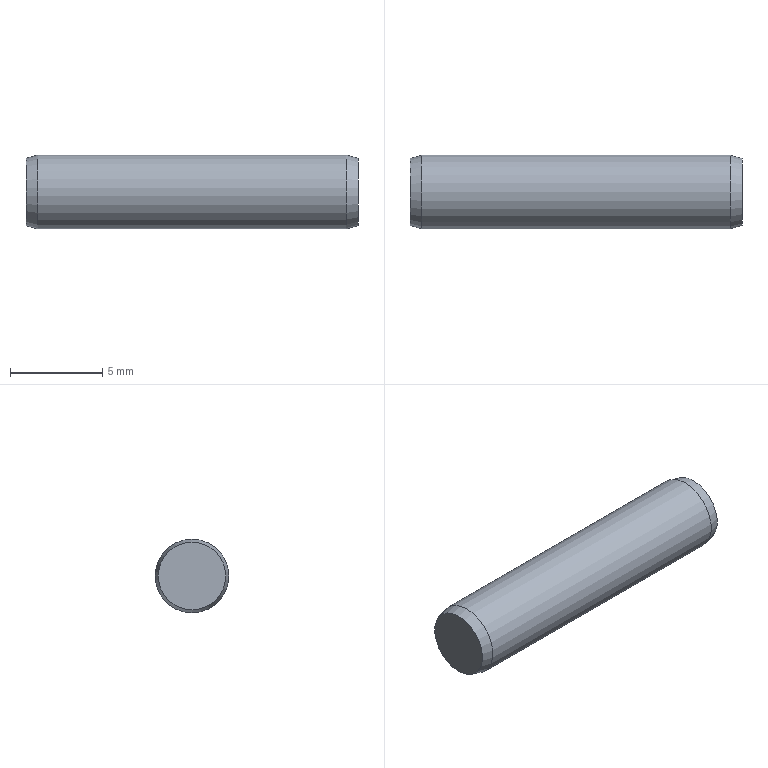Component | NX | DOWEL_PIN | 1 solid | 5 faces | box 18 x 4 x 4 mm | volume 225 mm3 | plane 2 | cone 2 | cylinder 1 | commonest cylinder face diameters 4 x1
STEP:
#1=CARTESIAN_POINT('',(0.,0.,0.));
#2=DIRECTION('',(0.,0.,1.));
#3=DIRECTION('',(1.,0.,0.));
#4=AXIS2_PLACEMENT_3D('',#1,#2,#3);
#5=CARTESIAN_POINT('',(36.5,-0.,-1.331));
#6=VERTEX_POINT('',#5);
#7=CARTESIAN_POINT('',(36.5,-0.,0.5));
#8=DIRECTION('',(1.,0.,0.));
#9=DIRECTION('',(0.,0.,-1.));
#10=AXIS2_PLACEMENT_3D('',#7,#8,#9);
#11=CIRCLE('',#10,1.831);
#12=CARTESIAN_POINT('',(36.5,-0.,0.5));
#13=DIRECTION('',(1.,0.,0.));
#14=DIRECTION('',(0.,0.,-1.));
#15=AXIS2_PLACEMENT_3D('',#12,#13,#14);
#16=PLANE('',#15);
#17=CARTESIAN_POINT('',(0.,0.));
#18=DIRECTION('',(1.,0.));
#19=AXIS2_PLACEMENT_2D('',#17,#18);
#20=CIRCLE('',#19,1.831);
#21=(GEOMETRIC_REPRESENTATION_CONTEXT(2)PARAMETRIC_REPRESENTATION_CONTEXT()REPRESENTATION_CONTEXT('',''));
#22=DEFINITIONAL_REPRESENTATION('',(#20),#21);
#23=PCURVE('',#16,#22);
#24=CARTESIAN_POINT('',(35.87,-0.,0.5));
#25=DIRECTION('',(-1.,0.,0.));
#26=DIRECTION('',(0.,0.,1.));
#27=AXIS2_PLACEMENT_3D('',#24,#25,#26);
#28=CONICAL_SURFACE('',#27,2.,0.2618);
#29=CARTESIAN_POINT('',(9.425,-0.63));
#30=DIRECTION('',(-1.,0.));
#31=VECTOR('',#30,1.);
#32=LINE('',#29,#31);
#33=(GEOMETRIC_REPRESENTATION_CONTEXT(2)PARAMETRIC_REPRESENTATION_CONTEXT()REPRESENTATION_CONTEXT('',''));
#34=DEFINITIONAL_REPRESENTATION('',(#32),#33);
#35=PCURVE('',#28,#34);
#36=SURFACE_CURVE('',#11,(#23,#35),.PCURVE_S1.);
#37=EDGE_CURVE('',#6,#6,#36,.T.);
#38=ORIENTED_EDGE('',*,*,#37,.T.);
#39=EDGE_LOOP('',(#38));
#40=FACE_BOUND('',#39,.T.);
#41=ADVANCED_FACE('',(#40),#16,.T.);
#42=CARTESIAN_POINT('',(18.5,-0.,2.331));
#43=VERTEX_POINT('',#42);
#44=CARTESIAN_POINT('',(18.5,-0.,0.5));
#45=DIRECTION('',(-1.,0.,0.));
#46=DIRECTION('',(0.,0.,1.));
#47=AXIS2_PLACEMENT_3D('',#44,#45,#46);
#48=CIRCLE('',#47,1.831);
#49=CARTESIAN_POINT('',(18.5,-0.,0.5));
#50=DIRECTION('',(-1.,0.,0.));
#51=DIRECTION('',(0.,0.,1.));
#52=AXIS2_PLACEMENT_3D('',#49,#50,#51);
#53=PLANE('',#52);
#54=CARTESIAN_POINT('',(0.,0.));
#55=DIRECTION('',(1.,0.));
#56=AXIS2_PLACEMENT_2D('',#54,#55);
#57=CIRCLE('',#56,1.831);
#58=(GEOMETRIC_REPRESENTATION_CONTEXT(2)PARAMETRIC_REPRESENTATION_CONTEXT()REPRESENTATION_CONTEXT('',''));
#59=DEFINITIONAL_REPRESENTATION('',(#57),#58);
#60=PCURVE('',#53,#59);
#61=CARTESIAN_POINT('',(19.13,-0.,0.5));
#62=DIRECTION('',(1.,0.,0.));
#63=DIRECTION('',(0.,0.,-1.));
#64=AXIS2_PLACEMENT_3D('',#61,#62,#63);
#65=CONICAL_SURFACE('',#64,2.,0.2618);
#66=CARTESIAN_POINT('',(9.425,-0.63));
#67=DIRECTION('',(-1.,0.));
#68=VECTOR('',#67,1.);
#69=LINE('',#66,#68);
#70=(GEOMETRIC_REPRESENTATION_CONTEXT(2)PARAMETRIC_REPRESENTATION_CONTEXT()REPRESENTATION_CONTEXT('',''));
#71=DEFINITIONAL_REPRESENTATION('',(#69),#70);
#72=PCURVE('',#65,#71);
#73=SURFACE_CURVE('',#48,(#60,#72),.PCURVE_S1.);
#74=EDGE_CURVE('',#43,#43,#73,.T.);
#75=ORIENTED_EDGE('',*,*,#74,.T.);
#76=EDGE_LOOP('',(#75));
#77=FACE_BOUND('',#76,.T.);
#78=ADVANCED_FACE('',(#77),#53,.T.);
#79=CARTESIAN_POINT('',(19.13,-0.,2.5));
#80=VERTEX_POINT('',#79);
#81=CARTESIAN_POINT('',(19.13,-0.,-1.5));
#82=VERTEX_POINT('',#81);
#83=CARTESIAN_POINT('',(19.13,-0.,0.5));
#84=DIRECTION('',(1.,0.,0.));
#85=DIRECTION('',(0.,0.,1.));
#86=AXIS2_PLACEMENT_3D('',#83,#84,#85);
#87=CIRCLE('',#86,2.);
#88=CARTESIAN_POINT('',(18.5,-0.,0.5));
#89=DIRECTION('',(1.,0.,0.));
#90=DIRECTION('',(0.,0.,-1.));
#91=AXIS2_PLACEMENT_3D('',#88,#89,#90);
#92=CYLINDRICAL_SURFACE('',#91,2.);
#93=CARTESIAN_POINT('',(3.142,0.63));
#94=DIRECTION('',(1.,0.));
#95=VECTOR('',#94,1.);
#96=LINE('',#93,#95);
#97=(GEOMETRIC_REPRESENTATION_CONTEXT(2)PARAMETRIC_REPRESENTATION_CONTEXT()REPRESENTATION_CONTEXT('',''));
#98=DEFINITIONAL_REPRESENTATION('',(#96),#97);
#99=PCURVE('',#92,#98);
#100=CARTESIAN_POINT('',(3.142,0.));
#101=DIRECTION('',(1.,0.));
#102=VECTOR('',#101,1.);
#103=LINE('',#100,#102);
#104=(GEOMETRIC_REPRESENTATION_CONTEXT(2)PARAMETRIC_REPRESENTATION_CONTEXT()REPRESENTATION_CONTEXT('',''));
#105=DEFINITIONAL_REPRESENTATION('',(#103),#104);
#106=PCURVE('',#65,#105);
#107=SURFACE_CURVE('',#87,(#99,#106),.PCURVE_S1.);
#108=EDGE_CURVE('',#80,#82,#107,.T.);
#109=ORIENTED_EDGE('',*,*,#108,.T.);
#110=CARTESIAN_POINT('',(35.87,-0.,-1.5));
#111=VERTEX_POINT('',#110);
#112=CARTESIAN_POINT('',(19.13,-0.,-1.5));
#113=CARTESIAN_POINT('',(35.87,-0.,-1.5));
#114=B_SPLINE_CURVE_WITH_KNOTS('',1,(#112,#113),.UNSPECIFIED.,.F.,.F.,(2,2),(0.63,17.37),.PIECEWISE_BEZIER_KNOTS.);
#115=CARTESIAN_POINT('',(6.283,0.));
#116=DIRECTION('',(0.,1.));
#117=VECTOR('',#116,1.);
#118=LINE('',#115,#117);
#119=(GEOMETRIC_REPRESENTATION_CONTEXT(2)PARAMETRIC_REPRESENTATION_CONTEXT()REPRESENTATION_CONTEXT('',''));
#120=DEFINITIONAL_REPRESENTATION('',(#118),#119);
#121=PCURVE('',#92,#120);
#122=CARTESIAN_POINT('',(0.,0.));
#123=DIRECTION('',(0.,1.));
#124=VECTOR('',#123,1.);
#125=LINE('',#122,#124);
#126=(GEOMETRIC_REPRESENTATION_CONTEXT(2)PARAMETRIC_REPRESENTATION_CONTEXT()REPRESENTATION_CONTEXT('',''));
#127=DEFINITIONAL_REPRESENTATION('',(#125),#126);
#128=PCURVE('',#92,#127);
#129=SEAM_CURVE('',#114,(#121,#128),.PCURVE_S1.);
#130=EDGE_CURVE('',#82,#111,#129,.T.);
#131=ORIENTED_EDGE('',*,*,#130,.T.);
#132=CARTESIAN_POINT('',(35.87,-0.,0.5));
#133=DIRECTION('',(-1.,0.,0.));
#134=DIRECTION('',(0.,0.,-1.));
#135=AXIS2_PLACEMENT_3D('',#132,#133,#134);
#136=CIRCLE('',#135,2.);
#137=CARTESIAN_POINT('',(6.283,17.37));
#138=DIRECTION('',(-1.,0.));
#139=VECTOR('',#138,1.);
#140=LINE('',#137,#139);
#141=(GEOMETRIC_REPRESENTATION_CONTEXT(2)PARAMETRIC_REPRESENTATION_CONTEXT()REPRESENTATION_CONTEXT('',''));
#142=DEFINITIONAL_REPRESENTATION('',(#140),#141);
#143=PCURVE('',#92,#142);
#144=CARTESIAN_POINT('',(3.142,0.));
#145=DIRECTION('',(1.,0.));
#146=VECTOR('',#145,1.);
#147=LINE('',#144,#146);
#148=(GEOMETRIC_REPRESENTATION_CONTEXT(2)PARAMETRIC_REPRESENTATION_CONTEXT()REPRESENTATION_CONTEXT('',''));
#149=DEFINITIONAL_REPRESENTATION('',(#147),#148);
#150=PCURVE('',#28,#149);
#151=SURFACE_CURVE('',#136,(#143,#150),.PCURVE_S1.);
#152=EDGE_CURVE('',#111,#111,#151,.T.);
#153=ORIENTED_EDGE('',*,*,#152,.T.);
#154=ORIENTED_EDGE('',*,*,#130,.F.);
#155=CARTESIAN_POINT('',(19.13,-0.,0.5));
#156=DIRECTION('',(1.,0.,0.));
#157=DIRECTION('',(0.,0.,1.));
#158=AXIS2_PLACEMENT_3D('',#155,#156,#157);
#159=CIRCLE('',#158,2.);
#160=CARTESIAN_POINT('',(-3.142,0.63));
#161=DIRECTION('',(1.,0.));
#162=VECTOR('',#161,1.);
#163=LINE('',#160,#162);
#164=(GEOMETRIC_REPRESENTATION_CONTEXT(2)PARAMETRIC_REPRESENTATION_CONTEXT()REPRESENTATION_CONTEXT('',''));
#165=DEFINITIONAL_REPRESENTATION('',(#163),#164);
#166=PCURVE('',#92,#165);
#167=CARTESIAN_POINT('',(3.142,0.));
#168=DIRECTION('',(1.,0.));
#169=VECTOR('',#168,1.);
#170=LINE('',#167,#169);
#171=(GEOMETRIC_REPRESENTATION_CONTEXT(2)PARAMETRIC_REPRESENTATION_CONTEXT()REPRESENTATION_CONTEXT('',''));
#172=DEFINITIONAL_REPRESENTATION('',(#170),#171);
#173=PCURVE('',#65,#172);
#174=SURFACE_CURVE('',#159,(#166,#173),.PCURVE_S1.);
#175=EDGE_CURVE('',#82,#80,#174,.T.);
#176=ORIENTED_EDGE('',*,*,#175,.T.);
#177=EDGE_LOOP('',(#109,#131,#153,#154,#176));
#178=FACE_BOUND('',#177,.T.);
#179=ADVANCED_FACE('',(#178),#92,.T.);
#180=ORIENTED_EDGE('',*,*,#74,.F.);
#181=CARTESIAN_POINT('',(18.5,-0.,2.331));
#182=CARTESIAN_POINT('',(19.13,-0.,2.5));
#183=B_SPLINE_CURVE_WITH_KNOTS('',1,(#181,#182),.UNSPECIFIED.,.F.,.F.,(2,2),(-0.6522,0.),.PIECEWISE_BEZIER_KNOTS.);
#184=CARTESIAN_POINT('',(9.425,0.));
#185=DIRECTION('',(0.,1.));
#186=VECTOR('',#185,1.);
#187=LINE('',#184,#186);
#188=(GEOMETRIC_REPRESENTATION_CONTEXT(2)PARAMETRIC_REPRESENTATION_CONTEXT()REPRESENTATION_CONTEXT('',''));
#189=DEFINITIONAL_REPRESENTATION('',(#187),#188);
#190=PCURVE('',#65,#189);
#191=CARTESIAN_POINT('',(3.142,0.));
#192=DIRECTION('',(0.,1.));
#193=VECTOR('',#192,1.);
#194=LINE('',#191,#193);
#195=(GEOMETRIC_REPRESENTATION_CONTEXT(2)PARAMETRIC_REPRESENTATION_CONTEXT()REPRESENTATION_CONTEXT('',''));
#196=DEFINITIONAL_REPRESENTATION('',(#194),#195);
#197=PCURVE('',#65,#196);
#198=SEAM_CURVE('',#183,(#190,#197),.PCURVE_S1.);
#199=EDGE_CURVE('',#43,#80,#198,.T.);
#200=ORIENTED_EDGE('',*,*,#199,.T.);
#201=ORIENTED_EDGE('',*,*,#175,.F.);
#202=ORIENTED_EDGE('',*,*,#108,.F.);
#203=ORIENTED_EDGE('',*,*,#199,.F.);
#204=EDGE_LOOP('',(#180,#200,#201,#202,#203));
#205=FACE_BOUND('',#204,.T.);
#206=ADVANCED_FACE('',(#205),#65,.T.);
#207=ORIENTED_EDGE('',*,*,#37,.F.);
#208=CARTESIAN_POINT('',(36.5,-0.,-1.331));
#209=CARTESIAN_POINT('',(35.87,-0.,-1.5));
#210=B_SPLINE_CURVE_WITH_KNOTS('',1,(#208,#209),.UNSPECIFIED.,.F.,.F.,(2,2),(-0.6522,0.),.PIECEWISE_BEZIER_KNOTS.);
#211=CARTESIAN_POINT('',(9.425,0.));
#212=DIRECTION('',(0.,1.));
#213=VECTOR('',#212,1.);
#214=LINE('',#211,#213);
#215=(GEOMETRIC_REPRESENTATION_CONTEXT(2)PARAMETRIC_REPRESENTATION_CONTEXT()REPRESENTATION_CONTEXT('',''));
#216=DEFINITIONAL_REPRESENTATION('',(#214),#215);
#217=PCURVE('',#28,#216);
#218=CARTESIAN_POINT('',(3.142,0.));
#219=DIRECTION('',(0.,1.));
#220=VECTOR('',#219,1.);
#221=LINE('',#218,#220);
#222=(GEOMETRIC_REPRESENTATION_CONTEXT(2)PARAMETRIC_REPRESENTATION_CONTEXT()REPRESENTATION_CONTEXT('',''));
#223=DEFINITIONAL_REPRESENTATION('',(#221),#222);
#224=PCURVE('',#28,#223);
#225=SEAM_CURVE('',#210,(#217,#224),.PCURVE_S1.);
#226=EDGE_CURVE('',#6,#111,#225,.T.);
#227=ORIENTED_EDGE('',*,*,#226,.T.);
#228=ORIENTED_EDGE('',*,*,#152,.F.);
#229=ORIENTED_EDGE('',*,*,#226,.F.);
#230=EDGE_LOOP('',(#207,#227,#228,#229));
#231=FACE_BOUND('',#230,.T.);
#232=ADVANCED_FACE('',(#231),#28,.T.);
#233=CLOSED_SHELL('',(#41,#78,#179,#206,#232));
#234=MANIFOLD_SOLID_BREP('',#233);
#235=(LENGTH_UNIT()NAMED_UNIT(*)SI_UNIT(.MILLI.,.METRE.));
#236=UNCERTAINTY_MEASURE_WITH_UNIT(LENGTH_MEASURE(0.00001),#235,'','');
#237=(NAMED_UNIT(*)PLANE_ANGLE_UNIT()SI_UNIT($,.RADIAN.));
#238=(NAMED_UNIT(*)SI_UNIT($,.STERADIAN.)SOLID_ANGLE_UNIT());
#239=(GEOMETRIC_REPRESENTATION_CONTEXT(3)GLOBAL_UNCERTAINTY_ASSIGNED_CONTEXT((#236))GLOBAL_UNIT_ASSIGNED_CONTEXT((#235,#237,#238))REPRESENTATION_CONTEXT('',''));
#240=ADVANCED_BREP_SHAPE_REPRESENTATION('',(#4,#234),#239);